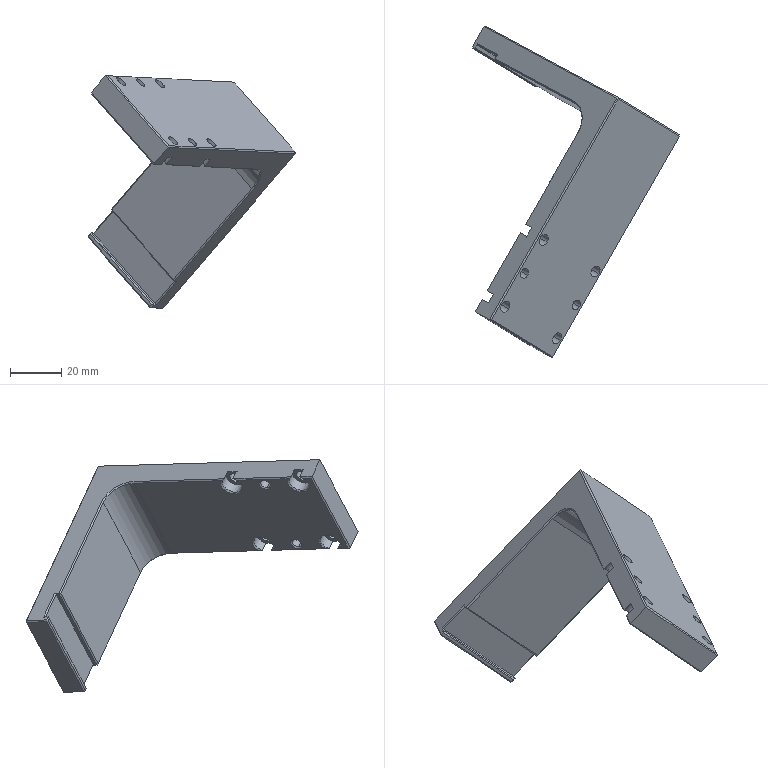Component | SolidWorks | 2z0-123-1 | 1 solid | 78 faces | box 80.59 x 129.27 x 90.54 mm | volume 68239 mm3 | plane 47 | cylinder 19 | cone 12 | commonest cylinder face diameters 4.5 x8 8 x6 4 x4 20 x1
build123d program:
from build123d import *

# Parameters (mm, degrees)
SKETCH1_W                                       = 85
SKETCH1_H                                       = 100
BOSS_EXTRUDE1_DEPTH                             = 40
SKETCH2_W                                       = 75
SKETCH2_H                                       = 90
CUT_EXTRUDE1_DEPTH                              = 77.852
FILLET1_R                                       = 10
M4_HEX_SOCKET_HEAD_CAP_SCREW_CBORE1_D           = 4.5
M4_HEX_SOCKET_HEAD_CAP_SCREW_CBORE1_CBORE_D     = 8
M4_HEX_SOCKET_HEAD_CAP_SCREW_CBORE1_CBORE_DEPTH = 4.4
SIZE_MM_DOWEL_PIN_HOLE1_D                       = 4
SIZE_MM_DOWEL_PIN_HOLE1_DEPTH                   = 10
SIZE_MM_DOWEL_PIN_HOLE1_TIP                     = 1.202
SKETCH8_W                                       = 12.7
SKETCH8_H                                       = 4
CUT_EXTRUDE2_DEPTH                              = 77.852
CHAMFER1_SIZE                                   = 0.5


with BuildPart() as part:
    # Sketch1 → Boss-Extrude1 (new body)
    with BuildSketch(Plane.XY):
        Rectangle(SKETCH1_W, SKETCH1_H)
    extrude(amount=BOSS_EXTRUDE1_DEPTH)

    # Sketch2 → Cut-Extrude1 (cut, through all)
    with BuildSketch(Plane.XY.offset(40)):
        with Locations((5, -5)):
            Rectangle(SKETCH2_W, SKETCH2_H)
    extrude(amount=-CUT_EXTRUDE1_DEPTH, mode=Mode.SUBTRACT)

    # Fillet1
    fillet1_edges = [part.edges().sort_by_distance(p)[0] for p in [
        (-32.5, 40, 20),
    ]]
    fillet(fillet1_edges, radius=FILLET1_R)

    # M4 Hex Socket Head Cap Screw CBORE1 (through all)
    with Locations(Plane(origin=(-32.5, -12.5, 36.5), x_dir=(0, 1, 0), z_dir=(1, 0, 0))):
        with Locations((0, 0), (-30, 0), (-30, -33), (0, -33)):
            CounterBoreHole(M4_HEX_SOCKET_HEAD_CAP_SCREW_CBORE1_D / 2, M4_HEX_SOCKET_HEAD_CAP_SCREW_CBORE1_CBORE_D / 2, M4_HEX_SOCKET_HEAD_CAP_SCREW_CBORE1_CBORE_DEPTH)

    # Size mm Dowel Pin Hole1
    with Locations(Plane(origin=(-32.5, 0, 0), x_dir=(0, 0, -1), z_dir=(1, 0, 0))):
        with Locations((-36.5, -27.5), (-3.5, -27.5)):
            Hole(SIZE_MM_DOWEL_PIN_HOLE1_D / 2, depth=SIZE_MM_DOWEL_PIN_HOLE1_DEPTH)
            with Locations((0, 0, -(SIZE_MM_DOWEL_PIN_HOLE1_DEPTH + SIZE_MM_DOWEL_PIN_HOLE1_TIP / 2))):  # 118° drill point
                Cone(0, SIZE_MM_DOWEL_PIN_HOLE1_D / 2, SIZE_MM_DOWEL_PIN_HOLE1_TIP, mode=Mode.SUBTRACT)

    # Sketch8 → Cut-Extrude2 (cut, through all)
    with BuildSketch(Plane.XY.offset(40)):
        with Locations((34, 40)):
            Rectangle(SKETCH8_W, SKETCH8_H)
    extrude(amount=-CUT_EXTRUDE2_DEPTH, mode=Mode.SUBTRACT)

    # Chamfer1
    chamfer1_edges = [part.edges().sort_by_distance(p)[0] for p in [
        (-42.5, 0, 40),
        (2.575, 40, 40),
        (2.575, 40, 0),
        (27.65, 40, 20),
        (40.35, 40, 20),
        (34, 42, 40),
        (34, 42, 0),
        (42.5, 45, 0),
        (42.5, 45, 40),
        (-32.5, -50, 20),
        (41.425, 40, 0),
        (42.5, 40, 20),
        (41.425, 40, 40),
        (-32.5, 9.718, 40),
        (-32.5, 9.718, 0),
        (-29.571, 37.071, 40),
        (-29.571, 37.071, 0),
        (-32.5, -27.5, 0),
        (-32.5, -12.5, 7.5),
        (-42.5, 0, 0),
        (-32.5, -47.218, 0),
        (0, 50, 0),
        (-32.5, -42.5, 7.5),
        (-32.5, -47.218, 40),
        (-32.5, -42.5, 32.5),
        (0, 50, 40),
        (-32.5, -27.5, 40),
        (-42.5, -50, 20),
        (-42.5, 50, 20),
        (42.5, 50, 20),
        (-32.5, -12.5, 32.5),
        (-32.5, -27.5, 1.5),
        (-32.5, -27.5, 34.5),
    ]]
    chamfer(chamfer1_edges, length=CHAMFER1_SIZE)


solid = part.part

# Placed as in the assembly
solid = solid.moved(Location((-51.495, -62.65, 114.861), (151.979, 37.728, -141.003)))